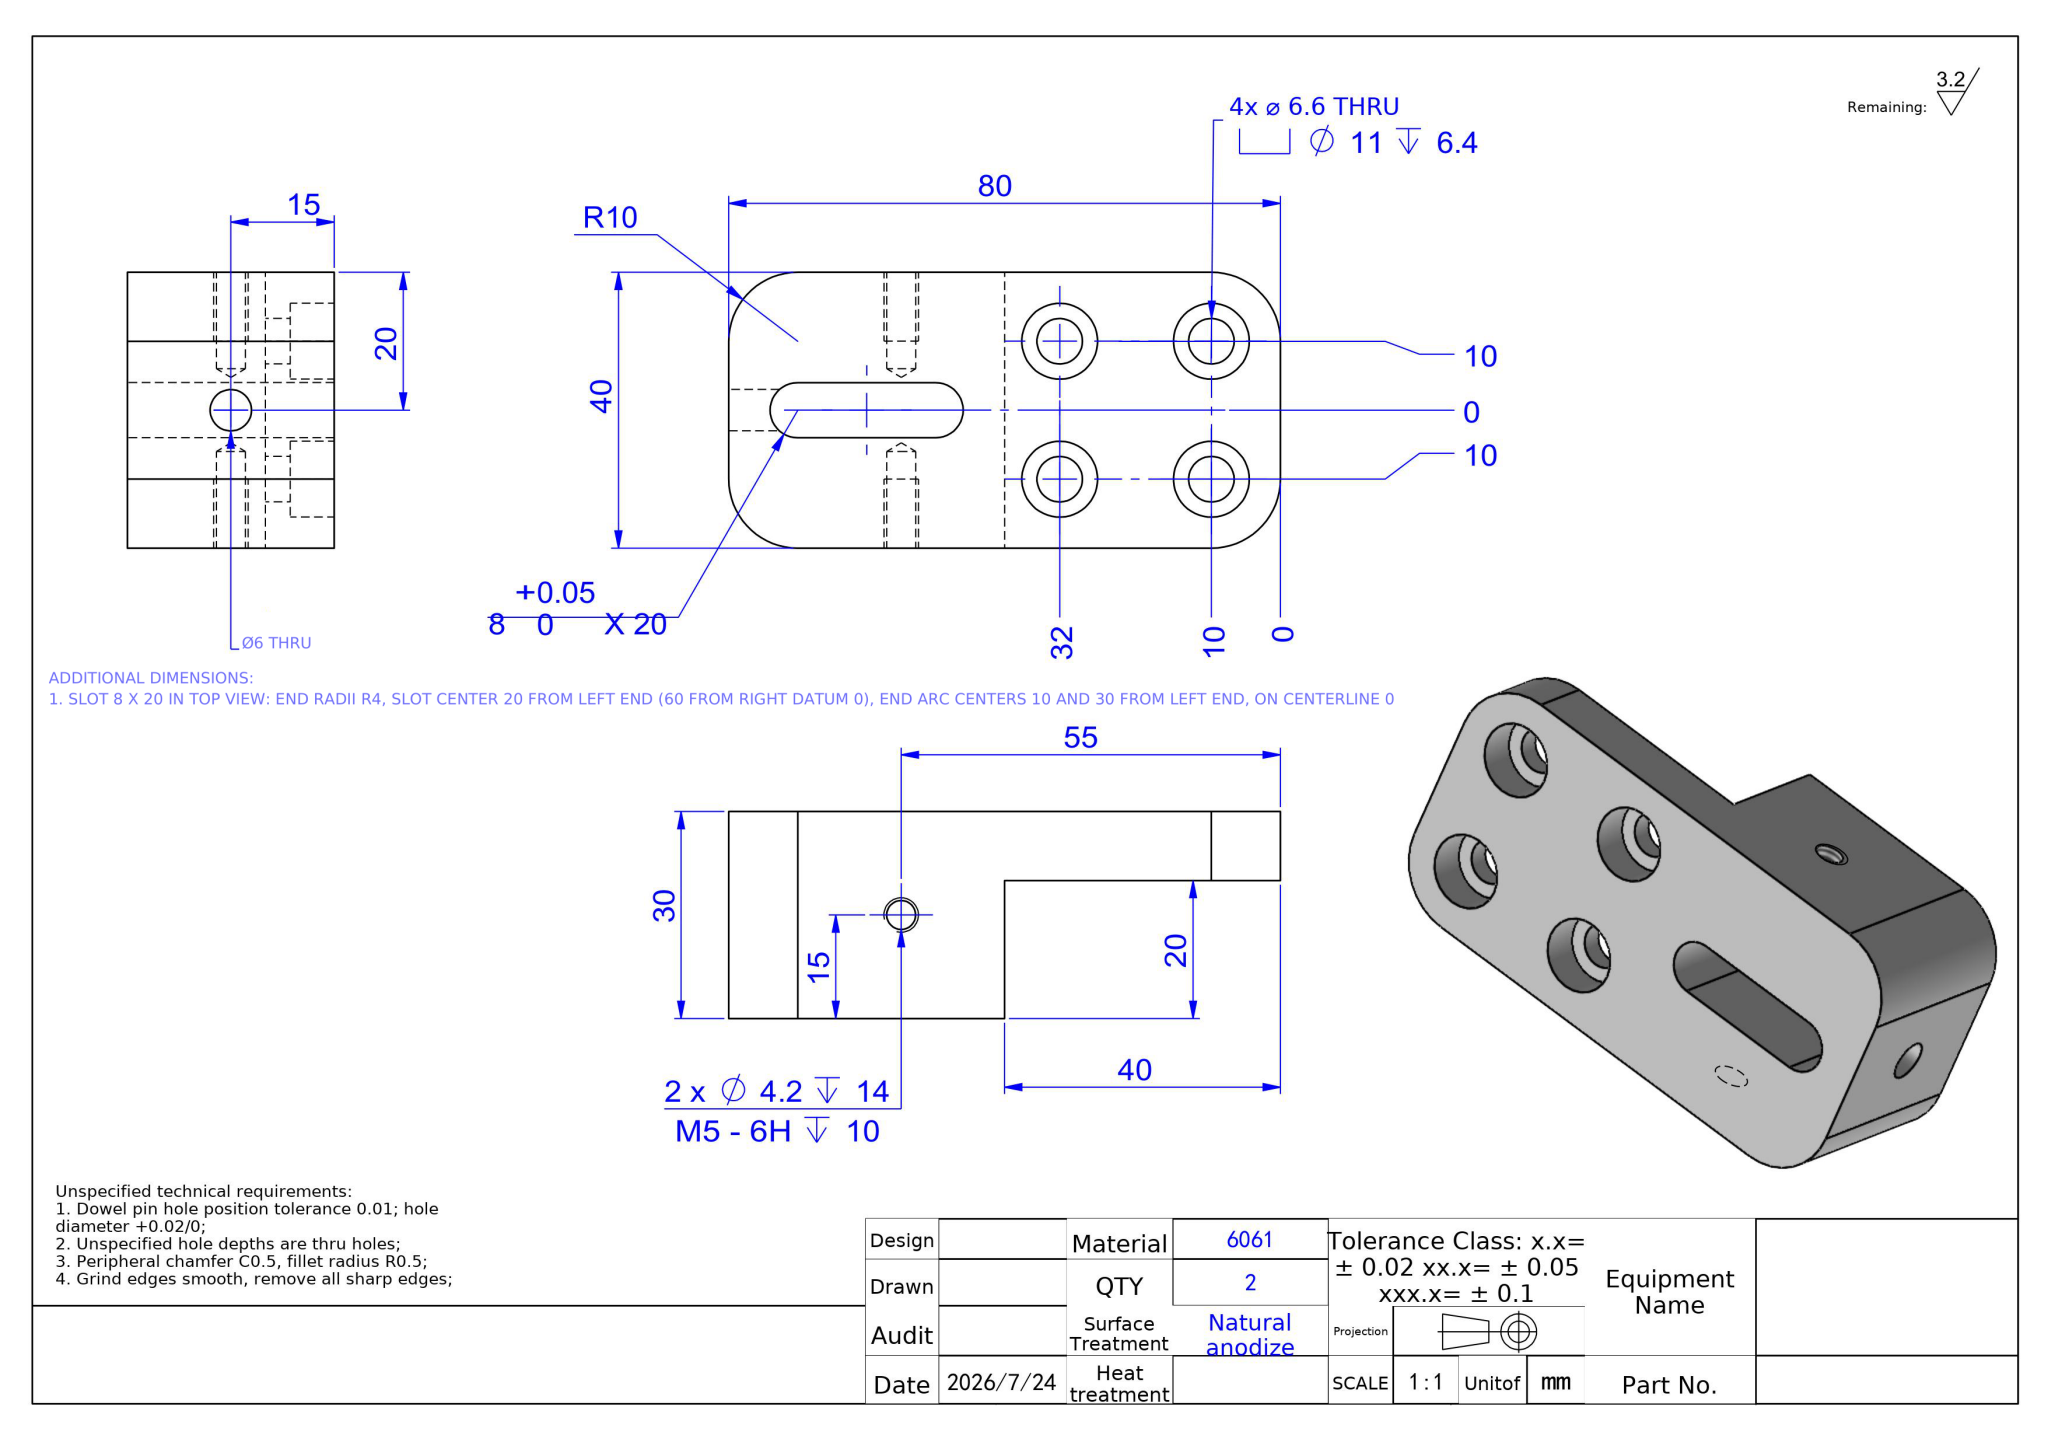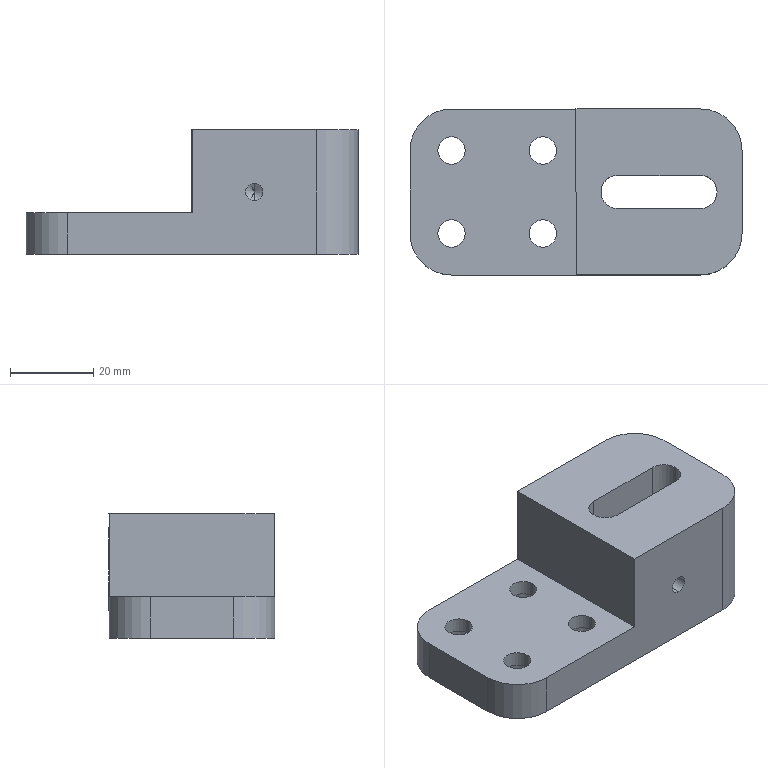Part | NX | mm | 1 solid | 47 faces | box 80 x 40 x 30 mm | volume 52472 mm3 | cylinder 29 | plane 14 | cone 4 | commonest cylinder face diameters 11 x8 6.6 x8 4.2 x4 20 x4 8 x3 6 x2